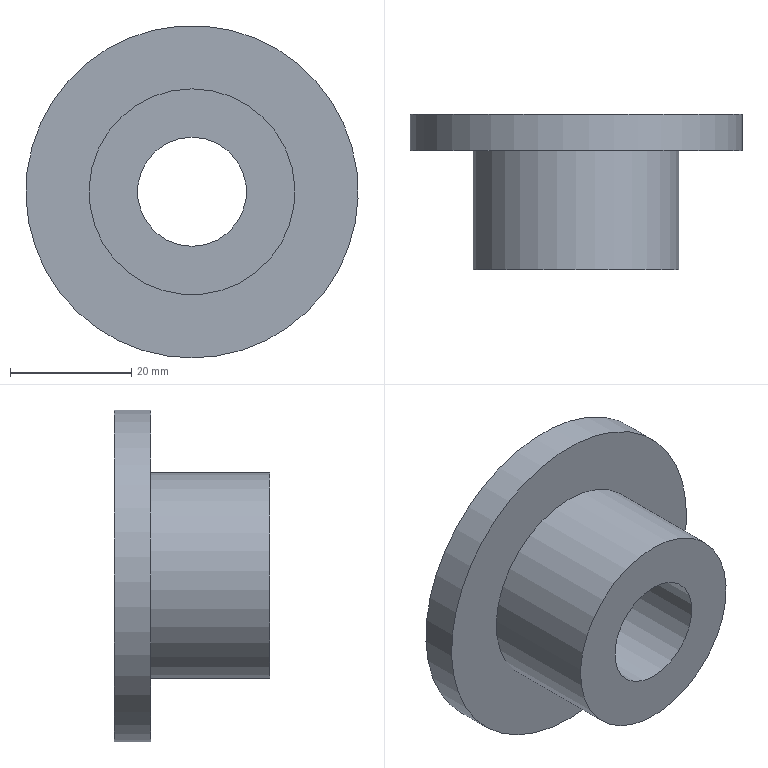Component | NX | SPRING_SLEEVE_2 | 1 solid | 6 faces | box 54.87 x 25.68 x 54.87 mm | volume 25525 mm3 | cylinder 3 | plane 3 | commonest cylinder face diameters 54.873 x1 34 x1 18 x1
STEP:
#1=CARTESIAN_POINT('',(0.,0.,0.));
#2=DIRECTION('',(0.,0.,1.));
#3=DIRECTION('',(1.,0.,0.));
#4=AXIS2_PLACEMENT_3D('',#1,#2,#3);
#5=CARTESIAN_POINT('',(0.,60.684,-27.437));
#6=VERTEX_POINT('',#5);
#7=CARTESIAN_POINT('',(0.,60.684,0.));
#8=DIRECTION('',(0.,-1.,0.));
#9=DIRECTION('',(0.,0.,-1.));
#10=AXIS2_PLACEMENT_3D('',#7,#8,#9);
#11=CIRCLE('',#10,27.437);
#12=CARTESIAN_POINT('',(0.,0.,0.));
#13=DIRECTION('',(0.,-1.,0.));
#14=DIRECTION('',(0.,0.,-1.));
#15=AXIS2_PLACEMENT_3D('',#12,#13,#14);
#16=CYLINDRICAL_SURFACE('',#15,27.437);
#17=CARTESIAN_POINT('',(0.,-60.684));
#18=DIRECTION('',(1.,0.));
#19=VECTOR('',#18,1.);
#20=LINE('',#17,#19);
#21=(GEOMETRIC_REPRESENTATION_CONTEXT(2)PARAMETRIC_REPRESENTATION_CONTEXT()REPRESENTATION_CONTEXT('',''));
#22=DEFINITIONAL_REPRESENTATION('',(#20),#21);
#23=PCURVE('',#16,#22);
#24=CARTESIAN_POINT('',(-27.437,60.684,0.));
#25=DIRECTION('',(0.,1.,0.));
#26=DIRECTION('',(0.,0.,1.));
#27=AXIS2_PLACEMENT_3D('',#24,#25,#26);
#28=PLANE('',#27);
#29=CARTESIAN_POINT('',(-27.437,27.437));
#30=CARTESIAN_POINT('',(-27.437,74.958));
#31=CARTESIAN_POINT('',(13.718,51.197));
#32=CARTESIAN_POINT('',(54.873,27.437));
#33=CARTESIAN_POINT('',(13.718,3.676));
#34=CARTESIAN_POINT('',(-27.437,-20.085));
#35=CARTESIAN_POINT('',(-27.437,27.437));
#36=(BOUNDED_CURVE()B_SPLINE_CURVE(2,(#29,#30,#31,#32,#33,#34,#35),.UNSPECIFIED.,.T.,.F.)B_SPLINE_CURVE_WITH_KNOTS((1,2,2,2,2,1),(-2.094,0.,2.094,4.189,6.283,8.378),.UNSPECIFIED.)CURVE()GEOMETRIC_REPRESENTATION_ITEM()RATIONAL_B_SPLINE_CURVE((1.,0.5,1.,0.5,1.,0.5,1.))REPRESENTATION_ITEM(''));
#37=(GEOMETRIC_REPRESENTATION_CONTEXT(2)PARAMETRIC_REPRESENTATION_CONTEXT()REPRESENTATION_CONTEXT('',''));
#38=DEFINITIONAL_REPRESENTATION('',(#36),#37);
#39=PCURVE('',#28,#38);
#40=SURFACE_CURVE('',#11,(#23,#39),.PCURVE_S1.);
#41=EDGE_CURVE('',#6,#6,#40,.T.);
#42=ORIENTED_EDGE('',*,*,#41,.F.);
#43=CARTESIAN_POINT('',(0.,66.684,-27.437));
#44=VERTEX_POINT('',#43);
#45=CARTESIAN_POINT('',(-0.,66.684,-27.437));
#46=CARTESIAN_POINT('',(-0.,60.684,-27.437));
#47=B_SPLINE_CURVE_WITH_KNOTS('',1,(#45,#46),.UNSPECIFIED.,.F.,.F.,(2,2),(-66.684,-60.684),.PIECEWISE_BEZIER_KNOTS.);
#48=CARTESIAN_POINT('',(0.,0.));
#49=DIRECTION('',(0.,1.));
#50=VECTOR('',#49,1.);
#51=LINE('',#48,#50);
#52=(GEOMETRIC_REPRESENTATION_CONTEXT(2)PARAMETRIC_REPRESENTATION_CONTEXT()REPRESENTATION_CONTEXT('',''));
#53=DEFINITIONAL_REPRESENTATION('',(#51),#52);
#54=PCURVE('',#16,#53);
#55=CARTESIAN_POINT('',(6.283,0.));
#56=DIRECTION('',(0.,1.));
#57=VECTOR('',#56,1.);
#58=LINE('',#55,#57);
#59=(GEOMETRIC_REPRESENTATION_CONTEXT(2)PARAMETRIC_REPRESENTATION_CONTEXT()REPRESENTATION_CONTEXT('',''));
#60=DEFINITIONAL_REPRESENTATION('',(#58),#59);
#61=PCURVE('',#16,#60);
#62=SEAM_CURVE('',#47,(#54,#61),.PCURVE_S1.);
#63=EDGE_CURVE('',#44,#6,#62,.T.);
#64=ORIENTED_EDGE('',*,*,#63,.F.);
#65=CARTESIAN_POINT('',(0.,66.684,0.));
#66=DIRECTION('',(0.,-1.,0.));
#67=DIRECTION('',(0.,0.,-1.));
#68=AXIS2_PLACEMENT_3D('',#65,#66,#67);
#69=CIRCLE('',#68,27.437);
#70=CARTESIAN_POINT('',(0.,-66.684));
#71=DIRECTION('',(1.,0.));
#72=VECTOR('',#71,1.);
#73=LINE('',#70,#72);
#74=(GEOMETRIC_REPRESENTATION_CONTEXT(2)PARAMETRIC_REPRESENTATION_CONTEXT()REPRESENTATION_CONTEXT('',''));
#75=DEFINITIONAL_REPRESENTATION('',(#73),#74);
#76=PCURVE('',#16,#75);
#77=CARTESIAN_POINT('',(-12.5,66.684,0.));
#78=DIRECTION('',(0.,-1.,0.));
#79=DIRECTION('',(0.,0.,-1.));
#80=AXIS2_PLACEMENT_3D('',#77,#78,#79);
#81=PLANE('',#80);
#82=CARTESIAN_POINT('',(0.,12.5));
#83=DIRECTION('',(1.,0.));
#84=AXIS2_PLACEMENT_2D('',#82,#83);
#85=CIRCLE('',#84,27.437);
#86=(GEOMETRIC_REPRESENTATION_CONTEXT(2)PARAMETRIC_REPRESENTATION_CONTEXT()REPRESENTATION_CONTEXT('',''));
#87=DEFINITIONAL_REPRESENTATION('',(#85),#86);
#88=PCURVE('',#81,#87);
#89=SURFACE_CURVE('',#69,(#76,#88),.PCURVE_S1.);
#90=EDGE_CURVE('',#44,#44,#89,.T.);
#91=ORIENTED_EDGE('',*,*,#90,.T.);
#92=ORIENTED_EDGE('',*,*,#63,.T.);
#93=EDGE_LOOP('',(#42,#64,#91,#92));
#94=FACE_BOUND('',#93,.T.);
#95=ADVANCED_FACE('',(#94),#16,.T.);
#96=CARTESIAN_POINT('',(0.,60.684,17.));
#97=VERTEX_POINT('',#96);
#98=CARTESIAN_POINT('',(0.,60.684,0.));
#99=DIRECTION('',(0.,-1.,0.));
#100=DIRECTION('',(0.,0.,1.));
#101=AXIS2_PLACEMENT_3D('',#98,#99,#100);
#102=CIRCLE('',#101,17.);
#103=CARTESIAN_POINT('',(17.,27.437));
#104=CARTESIAN_POINT('',(17.,-2.008));
#105=CARTESIAN_POINT('',(-8.5,12.714));
#106=CARTESIAN_POINT('',(-34.,27.437));
#107=CARTESIAN_POINT('',(-8.5,42.159));
#108=CARTESIAN_POINT('',(17.,56.881));
#109=CARTESIAN_POINT('',(17.,27.437));
#110=(BOUNDED_CURVE()B_SPLINE_CURVE(2,(#103,#104,#105,#106,#107,#108,#109),.UNSPECIFIED.,.T.,.F.)B_SPLINE_CURVE_WITH_KNOTS((1,2,2,2,2,1),(-2.094,0.,2.094,4.189,6.283,8.378),.UNSPECIFIED.)CURVE()GEOMETRIC_REPRESENTATION_ITEM()RATIONAL_B_SPLINE_CURVE((1.,0.5,1.,0.5,1.,0.5,1.))REPRESENTATION_ITEM(''));
#111=(GEOMETRIC_REPRESENTATION_CONTEXT(2)PARAMETRIC_REPRESENTATION_CONTEXT()REPRESENTATION_CONTEXT('',''));
#112=DEFINITIONAL_REPRESENTATION('',(#110),#111);
#113=PCURVE('',#28,#112);
#114=CARTESIAN_POINT('',(0.,0.,0.));
#115=DIRECTION('',(0.,-1.,0.));
#116=DIRECTION('',(0.,0.,-1.));
#117=AXIS2_PLACEMENT_3D('',#114,#115,#116);
#118=CYLINDRICAL_SURFACE('',#117,17.);
#119=CARTESIAN_POINT('',(3.142,-60.684));
#120=DIRECTION('',(1.,0.));
#121=VECTOR('',#120,1.);
#122=LINE('',#119,#121);
#123=(GEOMETRIC_REPRESENTATION_CONTEXT(2)PARAMETRIC_REPRESENTATION_CONTEXT()REPRESENTATION_CONTEXT('',''));
#124=DEFINITIONAL_REPRESENTATION('',(#122),#123);
#125=PCURVE('',#118,#124);
#126=SURFACE_CURVE('',#102,(#113,#125),.PCURVE_S1.);
#127=EDGE_CURVE('',#97,#97,#126,.T.);
#128=ORIENTED_EDGE('',*,*,#127,.F.);
#129=EDGE_LOOP('',(#128));
#130=FACE_BOUND('',#129,.T.);
#131=ORIENTED_EDGE('',*,*,#41,.T.);
#132=EDGE_LOOP('',(#131));
#133=FACE_BOUND('',#132,.T.);
#134=ADVANCED_FACE('',(#130,#133),#28,.F.);
#135=CARTESIAN_POINT('',(0.,41.001,17.));
#136=VERTEX_POINT('',#135);
#137=CARTESIAN_POINT('',(0.,41.001,0.));
#138=DIRECTION('',(0.,-1.,0.));
#139=DIRECTION('',(0.,0.,1.));
#140=AXIS2_PLACEMENT_3D('',#137,#138,#139);
#141=CIRCLE('',#140,17.);
#142=CARTESIAN_POINT('',(3.142,-41.001));
#143=DIRECTION('',(1.,0.));
#144=VECTOR('',#143,1.);
#145=LINE('',#142,#144);
#146=(GEOMETRIC_REPRESENTATION_CONTEXT(2)PARAMETRIC_REPRESENTATION_CONTEXT()REPRESENTATION_CONTEXT('',''));
#147=DEFINITIONAL_REPRESENTATION('',(#145),#146);
#148=PCURVE('',#118,#147);
#149=CARTESIAN_POINT('',(-17.456,41.001,0.));
#150=DIRECTION('',(0.,1.,0.));
#151=DIRECTION('',(0.,0.,1.));
#152=AXIS2_PLACEMENT_3D('',#149,#150,#151);
#153=PLANE('',#152);
#154=CARTESIAN_POINT('',(17.,17.456));
#155=CARTESIAN_POINT('',(17.,-11.989));
#156=CARTESIAN_POINT('',(-8.5,2.733));
#157=CARTESIAN_POINT('',(-34.,17.456));
#158=CARTESIAN_POINT('',(-8.5,32.178));
#159=CARTESIAN_POINT('',(17.,46.9));
#160=CARTESIAN_POINT('',(17.,17.456));
#161=(BOUNDED_CURVE()B_SPLINE_CURVE(2,(#154,#155,#156,#157,#158,#159,#160),.UNSPECIFIED.,.T.,.F.)B_SPLINE_CURVE_WITH_KNOTS((1,2,2,2,2,1),(-2.094,0.,2.094,4.189,6.283,8.378),.UNSPECIFIED.)CURVE()GEOMETRIC_REPRESENTATION_ITEM()RATIONAL_B_SPLINE_CURVE((1.,0.5,1.,0.5,1.,0.5,1.))REPRESENTATION_ITEM(''));
#162=(GEOMETRIC_REPRESENTATION_CONTEXT(2)PARAMETRIC_REPRESENTATION_CONTEXT()REPRESENTATION_CONTEXT('',''));
#163=DEFINITIONAL_REPRESENTATION('',(#161),#162);
#164=PCURVE('',#153,#163);
#165=SURFACE_CURVE('',#141,(#148,#164),.PCURVE_S1.);
#166=EDGE_CURVE('',#136,#136,#165,.T.);
#167=ORIENTED_EDGE('',*,*,#166,.F.);
#168=CARTESIAN_POINT('',(0.,60.684,17.));
#169=CARTESIAN_POINT('',(0.,41.001,17.));
#170=B_SPLINE_CURVE_WITH_KNOTS('',1,(#168,#169),.UNSPECIFIED.,.F.,.F.,(2,2),(-60.684,-41.001),.PIECEWISE_BEZIER_KNOTS.);
#171=CARTESIAN_POINT('',(3.142,0.));
#172=DIRECTION('',(0.,1.));
#173=VECTOR('',#172,1.);
#174=LINE('',#171,#173);
#175=(GEOMETRIC_REPRESENTATION_CONTEXT(2)PARAMETRIC_REPRESENTATION_CONTEXT()REPRESENTATION_CONTEXT('',''));
#176=DEFINITIONAL_REPRESENTATION('',(#174),#175);
#177=PCURVE('',#118,#176);
#178=CARTESIAN_POINT('',(9.425,0.));
#179=DIRECTION('',(0.,1.));
#180=VECTOR('',#179,1.);
#181=LINE('',#178,#180);
#182=(GEOMETRIC_REPRESENTATION_CONTEXT(2)PARAMETRIC_REPRESENTATION_CONTEXT()REPRESENTATION_CONTEXT('',''));
#183=DEFINITIONAL_REPRESENTATION('',(#181),#182);
#184=PCURVE('',#118,#183);
#185=SEAM_CURVE('',#170,(#177,#184),.PCURVE_S1.);
#186=EDGE_CURVE('',#97,#136,#185,.T.);
#187=ORIENTED_EDGE('',*,*,#186,.F.);
#188=ORIENTED_EDGE('',*,*,#127,.T.);
#189=ORIENTED_EDGE('',*,*,#186,.T.);
#190=EDGE_LOOP('',(#167,#187,#188,#189));
#191=FACE_BOUND('',#190,.T.);
#192=ADVANCED_FACE('',(#191),#118,.T.);
#193=CARTESIAN_POINT('',(0.,41.001,9.));
#194=VERTEX_POINT('',#193);
#195=CARTESIAN_POINT('',(0.,41.001,-9.));
#196=VERTEX_POINT('',#195);
#197=CARTESIAN_POINT('',(0.,41.001,0.));
#198=DIRECTION('',(0.,-1.,0.));
#199=DIRECTION('',(0.,0.,1.));
#200=AXIS2_PLACEMENT_3D('',#197,#198,#199);
#201=CIRCLE('',#200,9.);
#202=CARTESIAN_POINT('',(9.,17.456));
#203=CARTESIAN_POINT('',(9.,1.867));
#204=CARTESIAN_POINT('',(-4.5,9.661));
#205=CARTESIAN_POINT('',(-18.,17.456));
#206=CARTESIAN_POINT('',(-4.5,25.25));
#207=CARTESIAN_POINT('',(9.,33.044));
#208=CARTESIAN_POINT('',(9.,17.456));
#209=(BOUNDED_CURVE()B_SPLINE_CURVE(2,(#202,#203,#204,#205,#206,#207,#208),.UNSPECIFIED.,.T.,.F.)B_SPLINE_CURVE_WITH_KNOTS((1,2,2,2,2,1),(-2.094,0.,2.094,4.189,6.283,8.378),.UNSPECIFIED.)CURVE()GEOMETRIC_REPRESENTATION_ITEM()RATIONAL_B_SPLINE_CURVE((1.,0.5,1.,0.5,1.,0.5,1.))REPRESENTATION_ITEM(''));
#210=(GEOMETRIC_REPRESENTATION_CONTEXT(2)PARAMETRIC_REPRESENTATION_CONTEXT()REPRESENTATION_CONTEXT('',''));
#211=DEFINITIONAL_REPRESENTATION('',(#209),#210);
#212=PCURVE('',#153,#211);
#213=CARTESIAN_POINT('',(0.,87.,0.));
#214=DIRECTION('',(0.,-1.,0.));
#215=DIRECTION('',(0.,0.,-1.));
#216=AXIS2_PLACEMENT_3D('',#213,#214,#215);
#217=CYLINDRICAL_SURFACE('',#216,9.);
#218=CARTESIAN_POINT('',(3.142,45.999));
#219=DIRECTION('',(1.,0.));
#220=VECTOR('',#219,1.);
#221=LINE('',#218,#220);
#222=(GEOMETRIC_REPRESENTATION_CONTEXT(2)PARAMETRIC_REPRESENTATION_CONTEXT()REPRESENTATION_CONTEXT('',''));
#223=DEFINITIONAL_REPRESENTATION('',(#221),#222);
#224=PCURVE('',#217,#223);
#225=SURFACE_CURVE('',#201,(#212,#224),.PCURVE_S1.);
#226=EDGE_CURVE('',#194,#196,#225,.T.);
#227=ORIENTED_EDGE('',*,*,#226,.F.);
#228=CARTESIAN_POINT('',(0.,41.001,0.));
#229=DIRECTION('',(0.,-1.,0.));
#230=DIRECTION('',(0.,0.,1.));
#231=AXIS2_PLACEMENT_3D('',#228,#229,#230);
#232=CIRCLE('',#231,9.);
#233=CARTESIAN_POINT('',(9.,17.456));
#234=CARTESIAN_POINT('',(9.,1.867));
#235=CARTESIAN_POINT('',(-4.5,9.661));
#236=CARTESIAN_POINT('',(-18.,17.456));
#237=CARTESIAN_POINT('',(-4.5,25.25));
#238=CARTESIAN_POINT('',(9.,33.044));
#239=CARTESIAN_POINT('',(9.,17.456));
#240=(BOUNDED_CURVE()B_SPLINE_CURVE(2,(#233,#234,#235,#236,#237,#238,#239),.UNSPECIFIED.,.T.,.F.)B_SPLINE_CURVE_WITH_KNOTS((1,2,2,2,2,1),(-2.094,0.,2.094,4.189,6.283,8.378),.UNSPECIFIED.)CURVE()GEOMETRIC_REPRESENTATION_ITEM()RATIONAL_B_SPLINE_CURVE((1.,0.5,1.,0.5,1.,0.5,1.))REPRESENTATION_ITEM(''));
#241=(GEOMETRIC_REPRESENTATION_CONTEXT(2)PARAMETRIC_REPRESENTATION_CONTEXT()REPRESENTATION_CONTEXT('',''));
#242=DEFINITIONAL_REPRESENTATION('',(#240),#241);
#243=PCURVE('',#153,#242);
#244=CARTESIAN_POINT('',(-3.142,45.999));
#245=DIRECTION('',(1.,0.));
#246=VECTOR('',#245,1.);
#247=LINE('',#244,#246);
#248=(GEOMETRIC_REPRESENTATION_CONTEXT(2)PARAMETRIC_REPRESENTATION_CONTEXT()REPRESENTATION_CONTEXT('',''));
#249=DEFINITIONAL_REPRESENTATION('',(#247),#248);
#250=PCURVE('',#217,#249);
#251=SURFACE_CURVE('',#232,(#243,#250),.PCURVE_S1.);
#252=EDGE_CURVE('',#196,#194,#251,.T.);
#253=ORIENTED_EDGE('',*,*,#252,.F.);
#254=EDGE_LOOP('',(#227,#253));
#255=FACE_BOUND('',#254,.T.);
#256=ORIENTED_EDGE('',*,*,#166,.T.);
#257=EDGE_LOOP('',(#256));
#258=FACE_BOUND('',#257,.T.);
#259=ADVANCED_FACE('',(#255,#258),#153,.F.);
#260=CARTESIAN_POINT('',(0.,66.684,-9.));
#261=VERTEX_POINT('',#260);
#262=CARTESIAN_POINT('',(0.,66.684,0.));
#263=DIRECTION('',(0.,-1.,0.));
#264=DIRECTION('',(0.,0.,-1.));
#265=AXIS2_PLACEMENT_3D('',#262,#263,#264);
#266=CIRCLE('',#265,9.);
#267=CARTESIAN_POINT('',(0.,20.316));
#268=DIRECTION('',(1.,0.));
#269=VECTOR('',#268,1.);
#270=LINE('',#267,#269);
#271=(GEOMETRIC_REPRESENTATION_CONTEXT(2)PARAMETRIC_REPRESENTATION_CONTEXT()REPRESENTATION_CONTEXT('',''));
#272=DEFINITIONAL_REPRESENTATION('',(#270),#271);
#273=PCURVE('',#217,#272);
#274=CARTESIAN_POINT('',(0.,12.5));
#275=DIRECTION('',(1.,0.));
#276=AXIS2_PLACEMENT_2D('',#274,#275);
#277=CIRCLE('',#276,9.);
#278=(GEOMETRIC_REPRESENTATION_CONTEXT(2)PARAMETRIC_REPRESENTATION_CONTEXT()REPRESENTATION_CONTEXT('',''));
#279=DEFINITIONAL_REPRESENTATION('',(#277),#278);
#280=PCURVE('',#81,#279);
#281=SURFACE_CURVE('',#266,(#273,#280),.PCURVE_S1.);
#282=EDGE_CURVE('',#261,#261,#281,.T.);
#283=ORIENTED_EDGE('',*,*,#282,.T.);
#284=CARTESIAN_POINT('',(0.,66.684,-9.));
#285=CARTESIAN_POINT('',(0.,41.001,-9.));
#286=B_SPLINE_CURVE_WITH_KNOTS('',1,(#284,#285),.UNSPECIFIED.,.F.,.F.,(2,2),(20.316,45.999),.PIECEWISE_BEZIER_KNOTS.);
#287=CARTESIAN_POINT('',(6.283,0.));
#288=DIRECTION('',(0.,1.));
#289=VECTOR('',#288,1.);
#290=LINE('',#287,#289);
#291=(GEOMETRIC_REPRESENTATION_CONTEXT(2)PARAMETRIC_REPRESENTATION_CONTEXT()REPRESENTATION_CONTEXT('',''));
#292=DEFINITIONAL_REPRESENTATION('',(#290),#291);
#293=PCURVE('',#217,#292);
#294=CARTESIAN_POINT('',(0.,0.));
#295=DIRECTION('',(0.,1.));
#296=VECTOR('',#295,1.);
#297=LINE('',#294,#296);
#298=(GEOMETRIC_REPRESENTATION_CONTEXT(2)PARAMETRIC_REPRESENTATION_CONTEXT()REPRESENTATION_CONTEXT('',''));
#299=DEFINITIONAL_REPRESENTATION('',(#297),#298);
#300=PCURVE('',#217,#299);
#301=SEAM_CURVE('',#286,(#293,#300),.PCURVE_S1.);
#302=EDGE_CURVE('',#261,#196,#301,.T.);
#303=ORIENTED_EDGE('',*,*,#302,.T.);
#304=ORIENTED_EDGE('',*,*,#226,.F.);
#305=ORIENTED_EDGE('',*,*,#252,.F.);
#306=ORIENTED_EDGE('',*,*,#302,.F.);
#307=EDGE_LOOP('',(#283,#303,#304,#305,#306));
#308=FACE_BOUND('',#307,.F.);
#309=ADVANCED_FACE('',(#308),#217,.F.);
#310=ORIENTED_EDGE('',*,*,#90,.F.);
#311=EDGE_LOOP('',(#310));
#312=FACE_BOUND('',#311,.T.);
#313=ORIENTED_EDGE('',*,*,#282,.T.);
#314=EDGE_LOOP('',(#313));
#315=FACE_BOUND('',#314,.T.);
#316=ADVANCED_FACE('',(#312,#315),#81,.F.);
#317=CLOSED_SHELL('',(#95,#134,#192,#259,#309,#316));
#318=MANIFOLD_SOLID_BREP('',#317);
#319=(LENGTH_UNIT()NAMED_UNIT(*)SI_UNIT(.MILLI.,.METRE.));
#320=UNCERTAINTY_MEASURE_WITH_UNIT(LENGTH_MEASURE(0.000005),#319,'','');
#321=(NAMED_UNIT(*)PLANE_ANGLE_UNIT()SI_UNIT($,.RADIAN.));
#322=(NAMED_UNIT(*)SI_UNIT($,.STERADIAN.)SOLID_ANGLE_UNIT());
#323=(GEOMETRIC_REPRESENTATION_CONTEXT(3)GLOBAL_UNCERTAINTY_ASSIGNED_CONTEXT((#320))GLOBAL_UNIT_ASSIGNED_CONTEXT((#319,#321,#322))REPRESENTATION_CONTEXT('',''));
#324=ADVANCED_BREP_SHAPE_REPRESENTATION('',(#4,#318),#323);